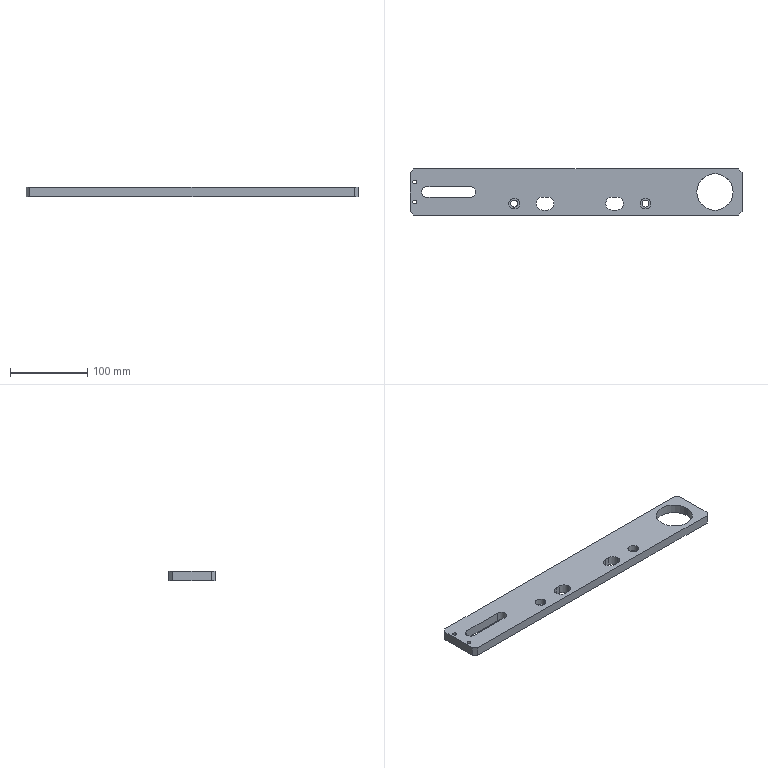Component | SolidWorks | -LowerSlideSleeveConnectionPlate02-1-1 | 1 solid | 41 faces | volume 265587 mm3 | cylinder 23 | plane 18 | commonest cylinder face diameters 14 x7 17 x6 5 x4 9 x4 47 x2